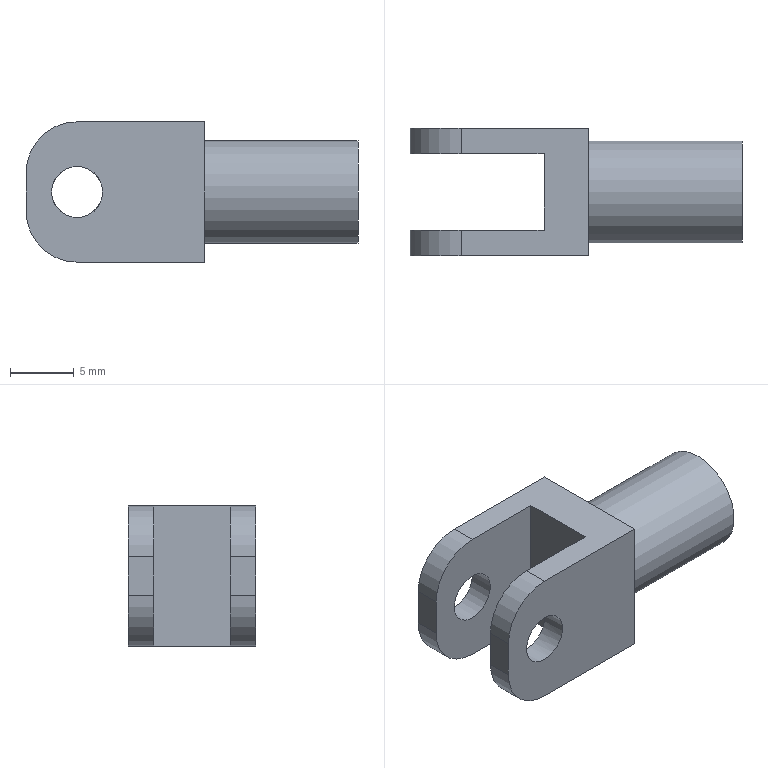Component | NX | CONNECTING_ROD_JOINT_2 | 1 solid | 20 faces | volume 1307 mm3 | plane 11 | cylinder 8 | cone 1 | commonest cylinder face diameters 8 x5 4 x2 3 x1